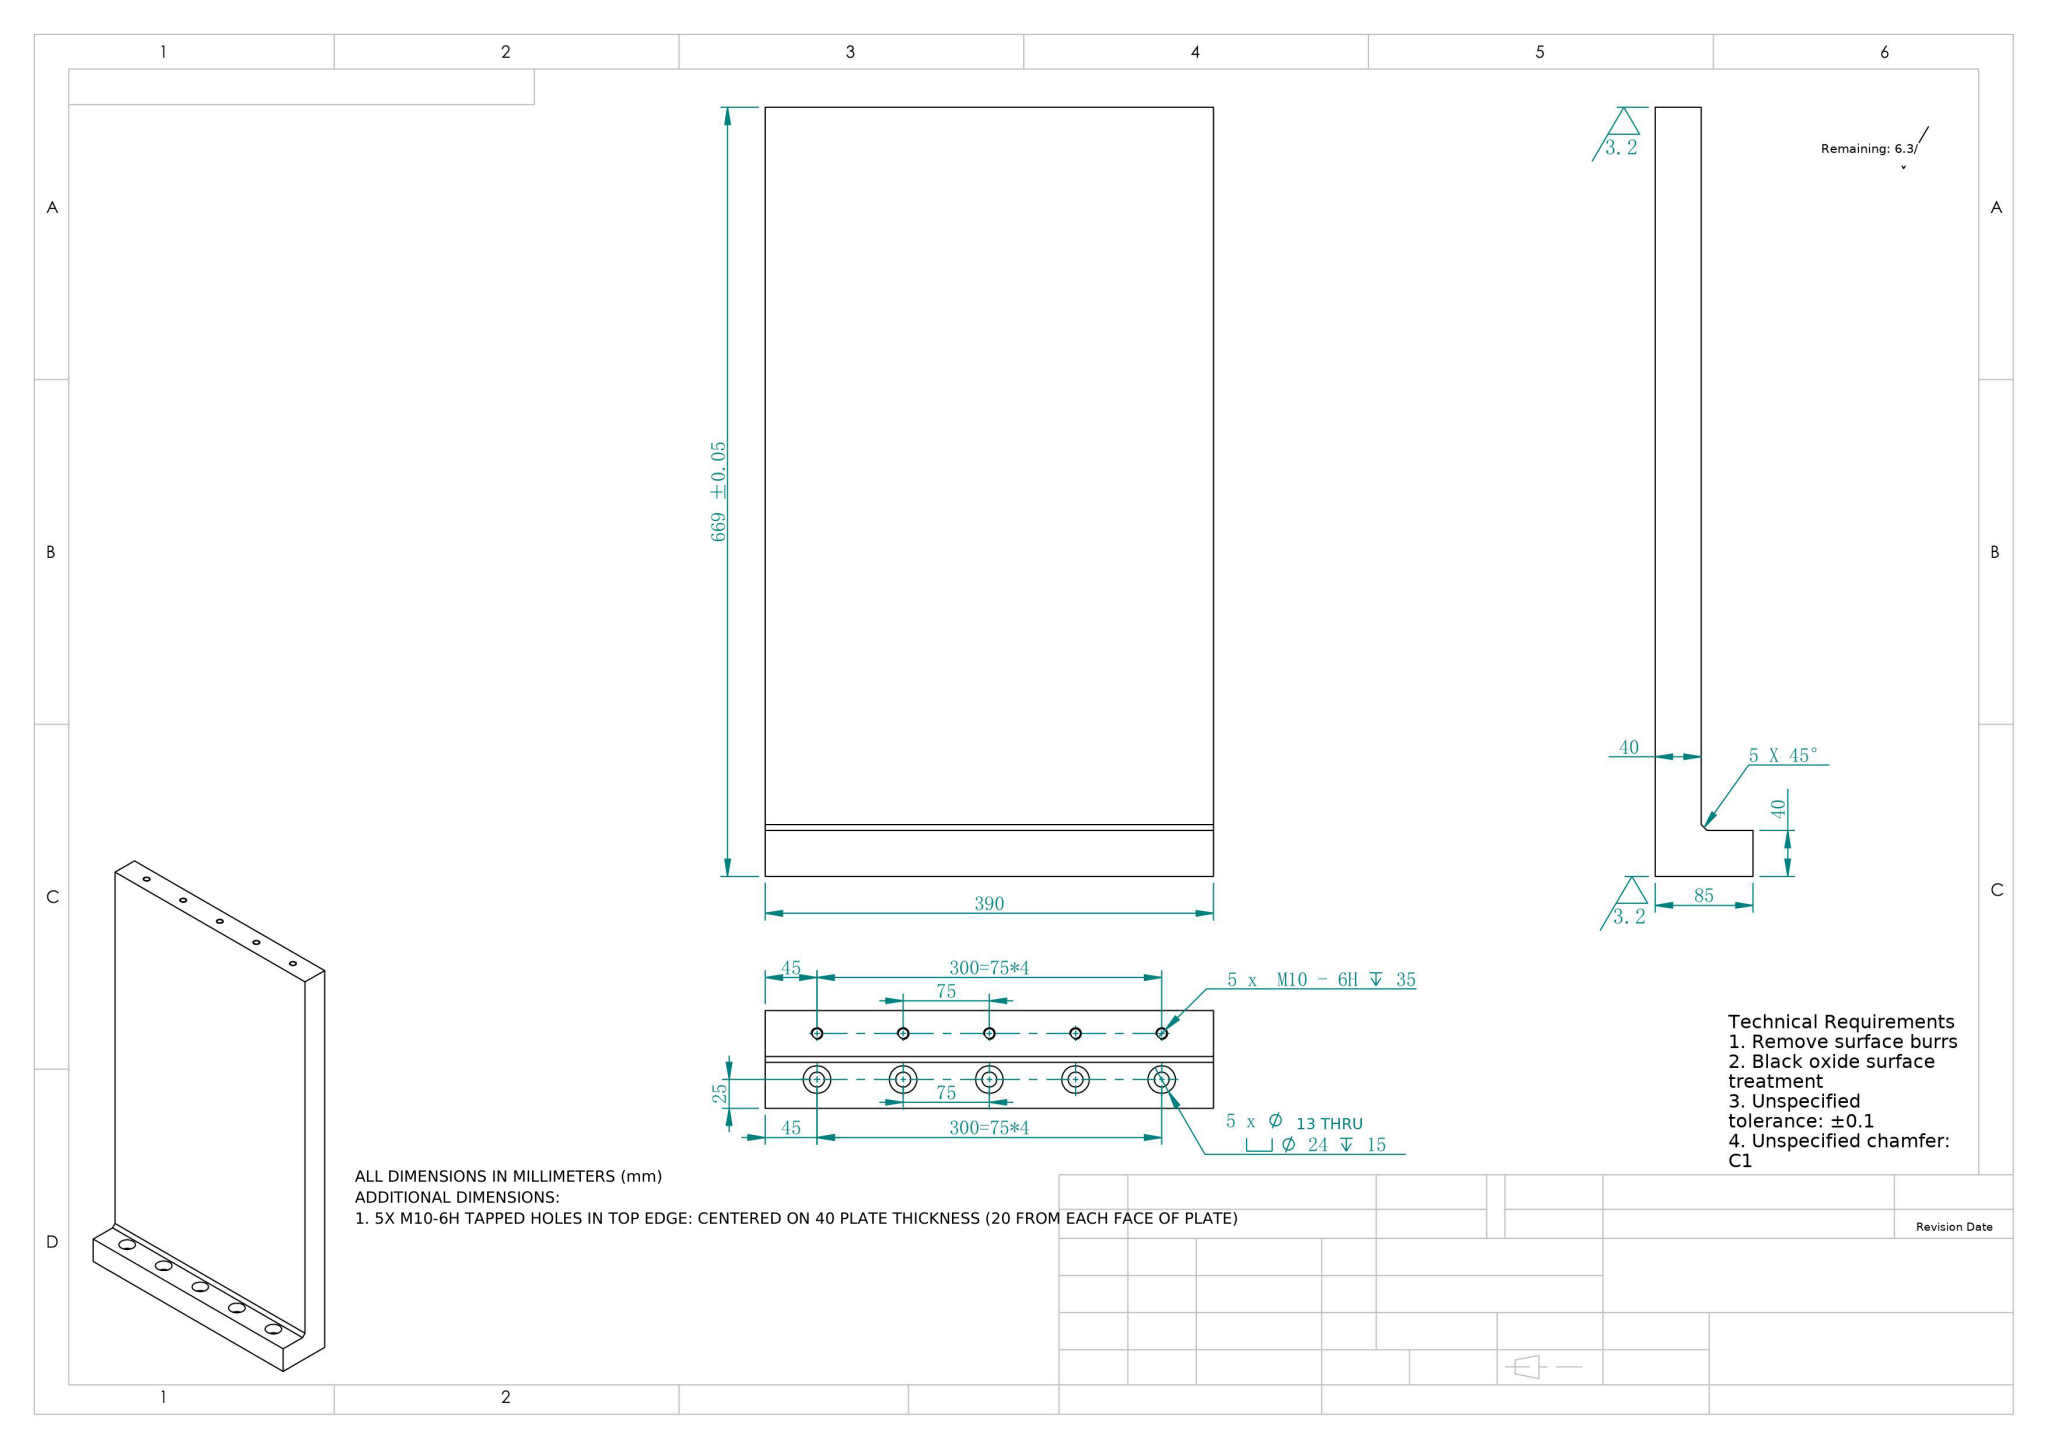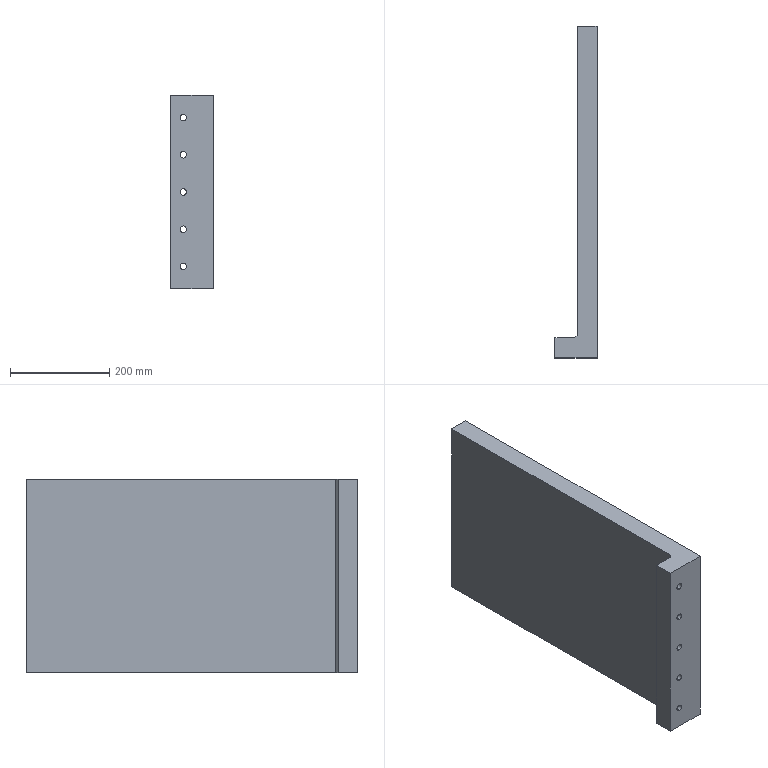Part | NX | mm | 1 solid | 54 faces | box 85 x 669 x 390 mm | volume 11082582 mm3 | cylinder 30 | plane 14 | cone 10 | commonest cylinder face diameters 8.5 x10 24 x10 13 x10